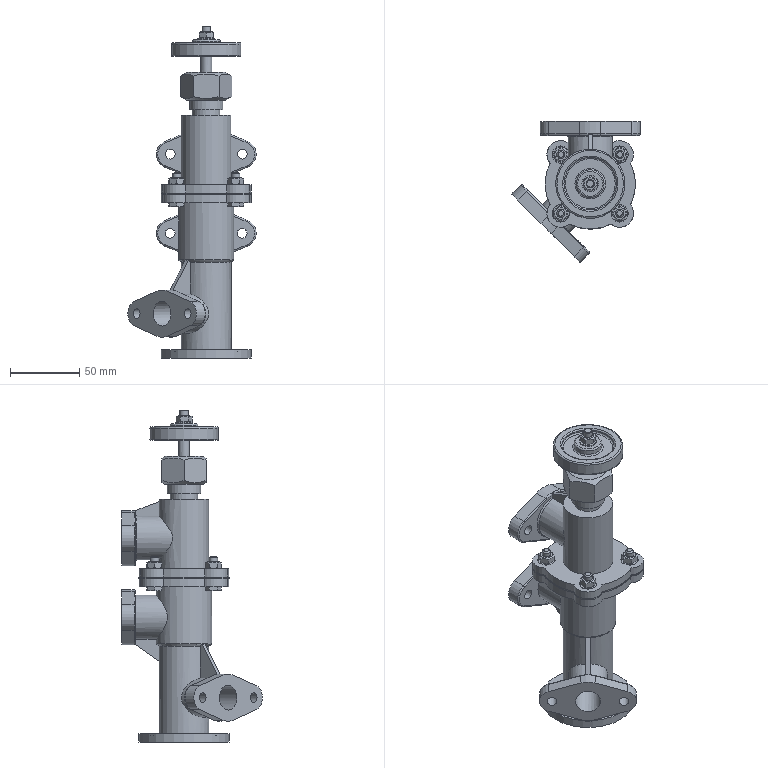Assembly | NX | mm | 24 component files | 24 solids | 429 faces | box 92.57 x 101.57 x 239.5 mm | volume 268416 mm3 | plane 185 | cylinder 154 | cone 64 | torus 26 | commonest cylinder face diameters 7 x22 6 x21 20 x21 65 x13 2 x12 12.5 x8 12 x7 36 x5
Bill of materials:
unnamed part 1 | 1 |  | Axisymmetric flanged sleeve: a short cylindrical collar above a thin circular flange, a slightly tapered body below it, and a chamfered lower tip, with an axial through bore.
unnamed part 2 | 5 |  | Flat plain annular ring with a concentric circular through hole and constant thickness.
unnamed part 3 | 1 |  | Multi-port tubular body: a vertical cylindrical tube with a four-lobed flange at one end and a round flange at the other, plus two side branches ending in oval two-hole flanges, one of which is joined to the tube by a web or gusset.
unnamed part 4 | 1 |  | Hexagonal prism with chamfered edges at both ends and a relatively small central through hole.
unnamed part 5 | 5 |  | Hexagonal prism with chamfered edges at both ends and a large central through hole.
unnamed part 6 | 1 |  | Slender stepped axisymmetric shaft with a double-cone collar partway along it, a larger cylindrical band above that, a reduced pin end at the top, and a stepped, tapered tip at the bottom.
unnamed part 7 | 4 |  | Hex-head shank part: a hexagonal head with a chamfered outer edge and a plain cylindrical shank with a chamfered free end.
unnamed part 8 | 1 |  | Thick circular disc with rounded edges, a raised central cylindrical boss with a square through hole, and a concentric annular groove or step on the top face.
unnamed part 9 | 1 |  | Stepped, flanged, tapered axisymmetric part: a top flange, a cylindrical section, a conical taper, a short smaller cylinder and a chamfered tip, with an internal conical cavity leading to a small through hole.
unnamed part 10 | 1 |  | Housing-like body: a four-lobed base flange with four holes, a vertical cylindrical body, and a smaller top neck with a chamfered rim and an axial bore. An angled side branch ends in an oval two-hole flange and is supported by a web.
unnamed part 11 | 1 |  | Flanged cylindrical sleeve (top-hat bushing form): a short larger-diameter flange over a slightly smaller cylindrical body, with a straight axial through bore.
unnamed part 12 | 1 |  | Thin flat plate with a four-lobed outline, a large central circular hole and four smaller holes, one in each lobe.
unnamed part 13 | 1 |  | Short axisymmetric cylindrical body with a central through-bore. Both ends are conical tapers that run from the outer cylindrical surface inward toward the bore edge, so the part has a double-chamfered, bead- or bushing-like profile.
Mates:
1. fix | lower_valve_body 1 component
2. touch align | upper_valve_body 1 face | lower_valve_body 1 face
3. touch align | upper_valve_body 1 face | lower_valve_body 1 face
4. touch align | gland 1 face | upper_valve_body 1 face
5. touch align | packing 1 face | lower_valve_body 1 face
6. concentric | packing 1 edge | upper_valve_body 1 edge
7. touch align | gland_nut 1 face | gland 1 face
8. parallel | gland_nut 1 face | upper_valve_body 1 face
9. concentric | small_nozzle 1 edge | lower_valve_body 1 edge
10. parallel | valve_stem 1 face | handwheel 1 face
11. concentric | handwheel 1 edge | valve_stem 1 edge
12. concentric | bolt_M6 4 edge | lower_valve_body 1 edge
13. concentric | washer_11 5 edge | upper_valve_body 1 edge
14. concentric | nut 5 edge | washer_11 5 edge
15. fix | assembly component
16. bond | bolt_M6 4 component | assembly component
17. bond | nut 5 component | assembly component
18. bond | washer_11 5 component | assembly component
19. bond | bolt_M6 3 component | assembly component
20. bond | nut 4 component | assembly component
21. bond | washer_11 4 component | assembly component
22. bond | bolt_M6 2 component | assembly component
23. bond | nut 3 component | assembly component
24. bond | washer_11 3 component | assembly component
25. bond | bolt_M6 1 component | assembly component
26. bond | nut 2 component | assembly component
27. bond | washer_11 2 component | assembly component
28. circular | assembly datumaxis | assembly cartesiancoordinatesystem | assembly cartesiancoordinatesystem | assembly cartesiancoordinatesystem | assembly cartesiancoordinatesystem
29. circular | assembly datumaxis | assembly cartesiancoordinatesystem | assembly cartesiancoordinatesystem | assembly cartesiancoordinatesystem | assembly cartesiancoordinatesystem
30. circular | assembly datumaxis | assembly cartesiancoordinatesystem | assembly cartesiancoordinatesystem | assembly cartesiancoordinatesystem | assembly cartesiancoordinatesystem
31. concentric | washer_11 1 edge | handwheel 1 edge
32. concentric | nut 1 edge | washer_11 1 edge
33. touch align | upper_valve_body 1 face | gasket 1 face
34. concentric | gasket 1 edge | lower_valve_body 1 edge
35. concentric | large_nozzle 1 edge | gasket 1 edge
36. fix | gland 1 component